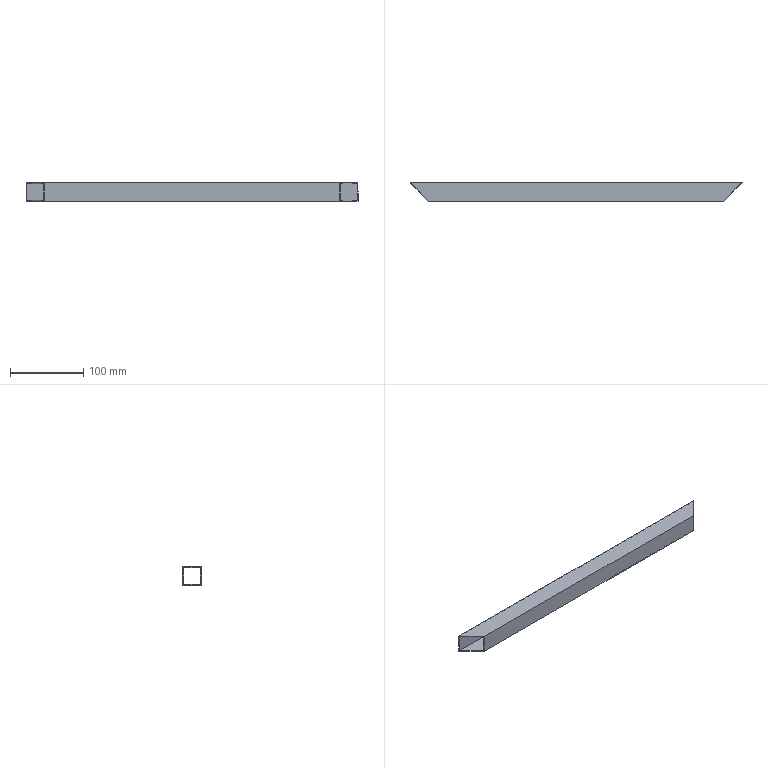Component | SolidWorks | dbj2-1_w8-1 | 1 solid | 10 faces | box 454 x 25 x 25 mm | volume 41184 mm3 | plane 10
build123d program:
from build123d import *

# Parameters (mm, degrees)
SKETCH1_W               = 25
SKETCH1_H               = 25
SKETCH1_W_2             = 23
SKETCH1_H_2             = 23
EXTRUDE_THIN1_DEPTH     = 454
CUT_EXTRUDE1_DEPTH      = 455.86
CUT_EXTRUDE1_DEPTH_BACK = 455.86
CUT_EXTRUDE2_DEPTH      = 455.86
CUT_EXTRUDE2_DEPTH_BACK = 455.86


with BuildPart() as part:
    # Sketch1 → Extrude-Thin1 (new body)
    with BuildSketch(Plane.XY):
        Rectangle(SKETCH1_W, SKETCH1_H)
        Rectangle(SKETCH1_W_2, SKETCH1_H_2, mode=Mode.SUBTRACT)
    extrude(amount=EXTRUDE_THIN1_DEPTH)

    # Sketch2 → Cut-Extrude1 (cut, two sides: drawn at the far end of the back side and taken through both)
    with BuildSketch(Plane(origin=(12.5, 0, 0), x_dir=(0, 0, -1), z_dir=(1, 0, 0)).offset(-CUT_EXTRUDE1_DEPTH_BACK)):
        Polygon((-1104.097, 662.597), (-454, 12.5), (-429, -12.5), (221.097, -662.597), (-1079.097, -1962.79), (-2404.29, -637.597), align=None)
    extrude(amount=CUT_EXTRUDE1_DEPTH + CUT_EXTRUDE1_DEPTH_BACK, mode=Mode.SUBTRACT)

    # Sketch3 → Cut-Extrude2 (cut, two sides: drawn at the far end of the back side and taken through both)
    with BuildSketch(Plane(origin=(12.5, 0, 0), x_dir=(0, 0, -1), z_dir=(1, 0, 0)).offset(-CUT_EXTRUDE2_DEPTH_BACK)):
        Polygon((650.097, 662.597), (0, 12.5), (-25, -12.5), (-675.097, -662.597), (625.097, -1962.79), (1950.29, -637.597), align=None)
    extrude(amount=CUT_EXTRUDE2_DEPTH + CUT_EXTRUDE2_DEPTH_BACK, mode=Mode.SUBTRACT)


solid = part.part

# Placed as in the assembly
solid = solid.moved(Location((-228, 714.25, -13.5), (0, 90, 0)))
STEP:
#1=COLOUR_RGB('',0.7922,0.8196,0.9333);
#2=FILL_AREA_STYLE_COLOUR('',#1);
#3=FILL_AREA_STYLE('',(#2));
#4=SURFACE_STYLE_FILL_AREA(#3);
#5=SURFACE_SIDE_STYLE('',(#4));
#6=SURFACE_STYLE_USAGE(.BOTH.,#5);
#7=PRESENTATION_STYLE_ASSIGNMENT((#6));
#8=CARTESIAN_POINT('',(7.913,27.628,-1.024));
#9=VERTEX_POINT('',#8);
#10=CARTESIAN_POINT('',(8.898,28.612,-1.024));
#11=VERTEX_POINT('',#10);
#12=CARTESIAN_POINT('',(-0.5315,19.183,-1.024));
#13=DIRECTION('',(0.7071,0.7071,0.));
#14=VECTOR('',#13,39.37);
#15=LINE('',#12,#14);
#16=EDGE_CURVE('',#9,#11,#15,.T.);
#17=ORIENTED_EDGE('',*,*,#16,.F.);
#18=CARTESIAN_POINT('',(-7.992,27.628,-1.024));
#19=VERTEX_POINT('',#18);
#20=CARTESIAN_POINT('',(-8.976,27.628,-1.024));
#21=DIRECTION('',(1.,0.,0.));
#22=VECTOR('',#21,39.37);
#23=LINE('',#20,#22);
#24=EDGE_CURVE('',#19,#9,#23,.T.);
#25=ORIENTED_EDGE('',*,*,#24,.F.);
#26=CARTESIAN_POINT('',(-8.976,28.612,-1.024));
#27=VERTEX_POINT('',#26);
#28=CARTESIAN_POINT('',(-8.484,28.12,-1.024));
#29=DIRECTION('',(-0.7071,0.7071,-0.));
#30=VECTOR('',#29,39.37);
#31=LINE('',#28,#30);
#32=EDGE_CURVE('',#19,#27,#31,.T.);
#33=ORIENTED_EDGE('',*,*,#32,.T.);
#34=CARTESIAN_POINT('',(-8.976,28.612,-1.024));
#35=DIRECTION('',(1.,0.,0.));
#36=VECTOR('',#35,39.37);
#37=LINE('',#34,#36);
#38=EDGE_CURVE('',#27,#11,#37,.T.);
#39=ORIENTED_EDGE('',*,*,#38,.T.);
#40=EDGE_LOOP('',(#17,#25,#33,#39));
#41=FACE_OUTER_BOUND('',#40,.T.);
#42=CARTESIAN_POINT('',(-8.976,27.628,-1.024));
#43=DIRECTION('',(-0.,0.,1.));
#44=DIRECTION('',(1.,0.,0.));
#45=AXIS2_PLACEMENT_3D('',#42,#43,#44);
#46=PLANE('',#45);
#47=ADVANCED_FACE('',(#41),#46,.F.);
#48=CARTESIAN_POINT('',(7.913,27.628,-0.03937));
#49=VERTEX_POINT('',#48);
#50=CARTESIAN_POINT('',(7.913,27.628,23.601));
#51=DIRECTION('',(0.,0.,-1.));
#52=VECTOR('',#51,39.37);
#53=LINE('',#50,#52);
#54=EDGE_CURVE('',#49,#9,#53,.T.);
#55=ORIENTED_EDGE('',*,*,#54,.F.);
#56=CARTESIAN_POINT('',(-7.992,27.628,-0.03937));
#57=VERTEX_POINT('',#56);
#58=CARTESIAN_POINT('',(-8.976,27.628,-0.03937));
#59=DIRECTION('',(1.,0.,0.));
#60=VECTOR('',#59,39.37);
#61=LINE('',#58,#60);
#62=EDGE_CURVE('',#57,#49,#61,.T.);
#63=ORIENTED_EDGE('',*,*,#62,.F.);
#64=CARTESIAN_POINT('',(-7.992,27.628,23.601));
#65=DIRECTION('',(0.,0.,-1.));
#66=VECTOR('',#65,39.37);
#67=LINE('',#64,#66);
#68=EDGE_CURVE('',#57,#19,#67,.T.);
#69=ORIENTED_EDGE('',*,*,#68,.T.);
#70=ORIENTED_EDGE('',*,*,#24,.T.);
#71=EDGE_LOOP('',(#55,#63,#69,#70));
#72=FACE_OUTER_BOUND('',#71,.T.);
#73=CARTESIAN_POINT('',(-8.976,27.628,-0.03937));
#74=DIRECTION('',(-0.,1.,-0.));
#75=DIRECTION('',(-1.,-0.,-0.));
#76=AXIS2_PLACEMENT_3D('',#73,#74,#75);
#77=PLANE('',#76);
#78=ADVANCED_FACE('',(#72),#77,.F.);
#79=CARTESIAN_POINT('',(8.898,28.612,-0.03937));
#80=VERTEX_POINT('',#79);
#81=CARTESIAN_POINT('',(-0.5315,19.183,-0.03937));
#82=DIRECTION('',(-0.7071,-0.7071,-0.));
#83=VECTOR('',#82,39.37);
#84=LINE('',#81,#83);
#85=EDGE_CURVE('',#80,#49,#84,.T.);
#86=ORIENTED_EDGE('',*,*,#85,.F.);
#87=CARTESIAN_POINT('',(-8.976,28.612,-0.03937));
#88=VERTEX_POINT('',#87);
#89=CARTESIAN_POINT('',(-8.976,28.612,-0.03937));
#90=DIRECTION('',(1.,0.,0.));
#91=VECTOR('',#90,39.37);
#92=LINE('',#89,#91);
#93=EDGE_CURVE('',#88,#80,#92,.T.);
#94=ORIENTED_EDGE('',*,*,#93,.F.);
#95=CARTESIAN_POINT('',(-8.484,28.12,-0.03937));
#96=DIRECTION('',(0.7071,-0.7071,0.));
#97=VECTOR('',#96,39.37);
#98=LINE('',#95,#97);
#99=EDGE_CURVE('',#88,#57,#98,.T.);
#100=ORIENTED_EDGE('',*,*,#99,.T.);
#101=ORIENTED_EDGE('',*,*,#62,.T.);
#102=EDGE_LOOP('',(#86,#94,#100,#101));
#103=FACE_OUTER_BOUND('',#102,.T.);
#104=CARTESIAN_POINT('',(-8.976,27.628,-0.03937));
#105=DIRECTION('',(0.,-0.,-1.));
#106=DIRECTION('',(-1.,-0.,-0.));
#107=AXIS2_PLACEMENT_3D('',#104,#105,#106);
#108=PLANE('',#107);
#109=ADVANCED_FACE('',(#103),#108,.F.);
#110=CARTESIAN_POINT('',(-8.031,27.667,-0.9843));
#111=VERTEX_POINT('',#110);
#112=CARTESIAN_POINT('',(7.953,27.667,-0.9843));
#113=VERTEX_POINT('',#112);
#114=CARTESIAN_POINT('',(-8.976,27.667,-0.9843));
#115=DIRECTION('',(1.,0.,0.));
#116=VECTOR('',#115,39.37);
#117=LINE('',#114,#116);
#118=EDGE_CURVE('',#111,#113,#117,.T.);
#119=ORIENTED_EDGE('',*,*,#118,.T.);
#120=CARTESIAN_POINT('',(8.858,28.573,-0.9843));
#121=VERTEX_POINT('',#120);
#122=CARTESIAN_POINT('',(-0.5315,19.183,-0.9843));
#123=DIRECTION('',(0.7071,0.7071,0.));
#124=VECTOR('',#123,39.37);
#125=LINE('',#122,#124);
#126=EDGE_CURVE('',#113,#121,#125,.T.);
#127=ORIENTED_EDGE('',*,*,#126,.T.);
#128=CARTESIAN_POINT('',(-8.937,28.573,-0.9843));
#129=VERTEX_POINT('',#128);
#130=CARTESIAN_POINT('',(-8.976,28.573,-0.9843));
#131=DIRECTION('',(1.,0.,0.));
#132=VECTOR('',#131,39.37);
#133=LINE('',#130,#132);
#134=EDGE_CURVE('',#129,#121,#133,.T.);
#135=ORIENTED_EDGE('',*,*,#134,.F.);
#136=CARTESIAN_POINT('',(-8.484,28.12,-0.9843));
#137=DIRECTION('',(-0.7071,0.7071,-0.));
#138=VECTOR('',#137,39.37);
#139=LINE('',#136,#138);
#140=EDGE_CURVE('',#111,#129,#139,.T.);
#141=ORIENTED_EDGE('',*,*,#140,.F.);
#142=EDGE_LOOP('',(#119,#127,#135,#141));
#143=FACE_OUTER_BOUND('',#142,.T.);
#144=CARTESIAN_POINT('',(-8.976,27.628,-0.9843));
#145=DIRECTION('',(-0.,0.,1.));
#146=DIRECTION('',(1.,0.,0.));
#147=AXIS2_PLACEMENT_3D('',#144,#145,#146);
#148=PLANE('',#147);
#149=ADVANCED_FACE('',(#143),#148,.T.);
#150=CARTESIAN_POINT('',(-8.031,27.667,-0.07874));
#151=VERTEX_POINT('',#150);
#152=CARTESIAN_POINT('',(7.953,27.667,-0.07874));
#153=VERTEX_POINT('',#152);
#154=CARTESIAN_POINT('',(-8.976,27.667,-0.07874));
#155=DIRECTION('',(1.,0.,0.));
#156=VECTOR('',#155,39.37);
#157=LINE('',#154,#156);
#158=EDGE_CURVE('',#151,#153,#157,.T.);
#159=ORIENTED_EDGE('',*,*,#158,.T.);
#160=CARTESIAN_POINT('',(7.953,27.667,-0.03937));
#161=DIRECTION('',(0.,0.,-1.));
#162=VECTOR('',#161,39.37);
#163=LINE('',#160,#162);
#164=EDGE_CURVE('',#153,#113,#163,.T.);
#165=ORIENTED_EDGE('',*,*,#164,.T.);
#166=ORIENTED_EDGE('',*,*,#118,.F.);
#167=CARTESIAN_POINT('',(-8.031,27.667,-0.03937));
#168=DIRECTION('',(0.,0.,-1.));
#169=VECTOR('',#168,39.37);
#170=LINE('',#167,#169);
#171=EDGE_CURVE('',#151,#111,#170,.T.);
#172=ORIENTED_EDGE('',*,*,#171,.F.);
#173=EDGE_LOOP('',(#159,#165,#166,#172));
#174=FACE_OUTER_BOUND('',#173,.T.);
#175=CARTESIAN_POINT('',(-8.976,27.667,-0.03937));
#176=DIRECTION('',(-0.,1.,-0.));
#177=DIRECTION('',(-1.,-0.,-0.));
#178=AXIS2_PLACEMENT_3D('',#175,#176,#177);
#179=PLANE('',#178);
#180=ADVANCED_FACE('',(#174),#179,.T.);
#181=CARTESIAN_POINT('',(-8.937,28.573,-0.07874));
#182=VERTEX_POINT('',#181);
#183=CARTESIAN_POINT('',(8.858,28.573,-0.07874));
#184=VERTEX_POINT('',#183);
#185=CARTESIAN_POINT('',(-8.976,28.573,-0.07874));
#186=DIRECTION('',(1.,0.,0.));
#187=VECTOR('',#186,39.37);
#188=LINE('',#185,#187);
#189=EDGE_CURVE('',#182,#184,#188,.T.);
#190=ORIENTED_EDGE('',*,*,#189,.T.);
#191=CARTESIAN_POINT('',(-0.5315,19.183,-0.07874));
#192=DIRECTION('',(-0.7071,-0.7071,-0.));
#193=VECTOR('',#192,39.37);
#194=LINE('',#191,#193);
#195=EDGE_CURVE('',#184,#153,#194,.T.);
#196=ORIENTED_EDGE('',*,*,#195,.T.);
#197=ORIENTED_EDGE('',*,*,#158,.F.);
#198=CARTESIAN_POINT('',(-8.484,28.12,-0.07874));
#199=DIRECTION('',(0.7071,-0.7071,0.));
#200=VECTOR('',#199,39.37);
#201=LINE('',#198,#200);
#202=EDGE_CURVE('',#182,#151,#201,.T.);
#203=ORIENTED_EDGE('',*,*,#202,.F.);
#204=EDGE_LOOP('',(#190,#196,#197,#203));
#205=FACE_OUTER_BOUND('',#204,.T.);
#206=CARTESIAN_POINT('',(-8.976,27.628,-0.07874));
#207=DIRECTION('',(0.,-0.,-1.));
#208=DIRECTION('',(-1.,-0.,-0.));
#209=AXIS2_PLACEMENT_3D('',#206,#207,#208);
#210=PLANE('',#209);
#211=ADVANCED_FACE('',(#205),#210,.T.);
#212=ORIENTED_EDGE('',*,*,#134,.T.);
#213=CARTESIAN_POINT('',(8.858,28.573,-0.03937));
#214=DIRECTION('',(-0.,0.,1.));
#215=VECTOR('',#214,39.37);
#216=LINE('',#213,#215);
#217=EDGE_CURVE('',#121,#184,#216,.T.);
#218=ORIENTED_EDGE('',*,*,#217,.T.);
#219=ORIENTED_EDGE('',*,*,#189,.F.);
#220=CARTESIAN_POINT('',(-8.937,28.573,-0.03937));
#221=DIRECTION('',(-0.,0.,1.));
#222=VECTOR('',#221,39.37);
#223=LINE('',#220,#222);
#224=EDGE_CURVE('',#129,#182,#223,.T.);
#225=ORIENTED_EDGE('',*,*,#224,.F.);
#226=EDGE_LOOP('',(#212,#218,#219,#225));
#227=FACE_OUTER_BOUND('',#226,.T.);
#228=CARTESIAN_POINT('',(-8.976,28.573,-0.03937));
#229=DIRECTION('',(0.,-1.,0.));
#230=DIRECTION('',(-0.,0.,1.));
#231=AXIS2_PLACEMENT_3D('',#228,#229,#230);
#232=PLANE('',#231);
#233=ADVANCED_FACE('',(#227),#232,.T.);
#234=CARTESIAN_POINT('',(8.898,28.612,-0.03937));
#235=DIRECTION('',(0.,-0.,-1.));
#236=VECTOR('',#235,39.37);
#237=LINE('',#234,#236);
#238=EDGE_CURVE('',#80,#11,#237,.T.);
#239=ORIENTED_EDGE('',*,*,#238,.T.);
#240=ORIENTED_EDGE('',*,*,#38,.F.);
#241=CARTESIAN_POINT('',(-8.976,28.612,-0.03937));
#242=DIRECTION('',(0.,-0.,-1.));
#243=VECTOR('',#242,39.37);
#244=LINE('',#241,#243);
#245=EDGE_CURVE('',#88,#27,#244,.T.);
#246=ORIENTED_EDGE('',*,*,#245,.F.);
#247=ORIENTED_EDGE('',*,*,#93,.T.);
#248=EDGE_LOOP('',(#239,#240,#246,#247));
#249=FACE_OUTER_BOUND('',#248,.T.);
#250=CARTESIAN_POINT('',(-8.976,28.612,-0.03937));
#251=DIRECTION('',(0.,-1.,0.));
#252=DIRECTION('',(-0.,0.,1.));
#253=AXIS2_PLACEMENT_3D('',#250,#251,#252);
#254=PLANE('',#253);
#255=ADVANCED_FACE('',(#249),#254,.F.);
#256=ORIENTED_EDGE('',*,*,#171,.T.);
#257=ORIENTED_EDGE('',*,*,#140,.T.);
#258=ORIENTED_EDGE('',*,*,#224,.T.);
#259=ORIENTED_EDGE('',*,*,#202,.T.);
#260=EDGE_LOOP('',(#256,#257,#258,#259));
#261=FACE_BOUND('',#260,.T.);
#262=ORIENTED_EDGE('',*,*,#32,.F.);
#263=ORIENTED_EDGE('',*,*,#68,.F.);
#264=ORIENTED_EDGE('',*,*,#99,.F.);
#265=ORIENTED_EDGE('',*,*,#245,.T.);
#266=EDGE_LOOP('',(#262,#263,#264,#265));
#267=FACE_OUTER_BOUND('',#266,.T.);
#268=CARTESIAN_POINT('',(-8.976,28.612,23.601));
#269=DIRECTION('',(0.7071,0.7071,0.));
#270=DIRECTION('',(-0.7071,0.7071,-0.));
#271=AXIS2_PLACEMENT_3D('',#268,#269,#270);
#272=PLANE('',#271);
#273=ADVANCED_FACE('',(#261,#267),#272,.F.);
#274=ORIENTED_EDGE('',*,*,#126,.F.);
#275=ORIENTED_EDGE('',*,*,#164,.F.);
#276=ORIENTED_EDGE('',*,*,#195,.F.);
#277=ORIENTED_EDGE('',*,*,#217,.F.);
#278=EDGE_LOOP('',(#274,#275,#276,#277));
#279=FACE_BOUND('',#278,.T.);
#280=ORIENTED_EDGE('',*,*,#54,.T.);
#281=ORIENTED_EDGE('',*,*,#16,.T.);
#282=ORIENTED_EDGE('',*,*,#238,.F.);
#283=ORIENTED_EDGE('',*,*,#85,.T.);
#284=EDGE_LOOP('',(#280,#281,#282,#283));
#285=FACE_OUTER_BOUND('',#284,.T.);
#286=CARTESIAN_POINT('',(8.898,28.612,23.601));
#287=DIRECTION('',(0.7071,-0.7071,0.));
#288=DIRECTION('',(0.7071,0.7071,0.));
#289=AXIS2_PLACEMENT_3D('',#286,#287,#288);
#290=PLANE('',#289);
#291=ADVANCED_FACE('',(#279,#285),#290,.T.);
#292=CLOSED_SHELL('',(#47,#78,#109,#149,#180,#211,#233,#255,#273,#291));
#293=MANIFOLD_SOLID_BREP('',#292);
#294=STYLED_ITEM('',(#7),#293);
#295=(LENGTH_UNIT()NAMED_UNIT(*)SI_UNIT($,.METRE.));
#296=LENGTH_MEASURE_WITH_UNIT(LENGTH_MEASURE(0.0254),#295);
#297=DIMENSIONAL_EXPONENTS(1.,0.,0.,0.,0.,0.,0.);
#298=(CONVERSION_BASED_UNIT('',#296)LENGTH_UNIT()NAMED_UNIT(#297));
#299=UNCERTAINTY_MEASURE_WITH_UNIT(LENGTH_MEASURE(0.00001),#298,'','');
#300=(NAMED_UNIT(*)PLANE_ANGLE_UNIT()SI_UNIT($,.RADIAN.));
#301=(NAMED_UNIT(*)SI_UNIT($,.STERADIAN.)SOLID_ANGLE_UNIT());
#302=(GEOMETRIC_REPRESENTATION_CONTEXT(3)GLOBAL_UNCERTAINTY_ASSIGNED_CONTEXT((#299))GLOBAL_UNIT_ASSIGNED_CONTEXT((#298,#300,#301))REPRESENTATION_CONTEXT('',''));
#303=MECHANICAL_DESIGN_GEOMETRIC_PRESENTATION_REPRESENTATION('',(#294),#302);
#304=PRESENTATION_LAYER_ASSIGNMENT('','',(#294));
#305=CARTESIAN_POINT('',(0.,0.,0.));
#306=DIRECTION('',(0.,0.,1.));
#307=DIRECTION('',(1.,0.,0.));
#308=AXIS2_PLACEMENT_3D('',#305,#306,#307);
#309=(LENGTH_UNIT()NAMED_UNIT(*)SI_UNIT($,.METRE.));
#310=LENGTH_MEASURE_WITH_UNIT(LENGTH_MEASURE(0.0254),#309);
#311=DIMENSIONAL_EXPONENTS(1.,0.,0.,0.,0.,0.,0.);
#312=(CONVERSION_BASED_UNIT('',#310)LENGTH_UNIT()NAMED_UNIT(#311));
#313=UNCERTAINTY_MEASURE_WITH_UNIT(LENGTH_MEASURE(0.00001),#312,'','');
#314=(NAMED_UNIT(*)PLANE_ANGLE_UNIT()SI_UNIT($,.RADIAN.));
#315=(NAMED_UNIT(*)SI_UNIT($,.STERADIAN.)SOLID_ANGLE_UNIT());
#316=(GEOMETRIC_REPRESENTATION_CONTEXT(3)GLOBAL_UNCERTAINTY_ASSIGNED_CONTEXT((#313))GLOBAL_UNIT_ASSIGNED_CONTEXT((#312,#314,#315))REPRESENTATION_CONTEXT('',''));
#317=ADVANCED_BREP_SHAPE_REPRESENTATION('',(#293,#308),#316);